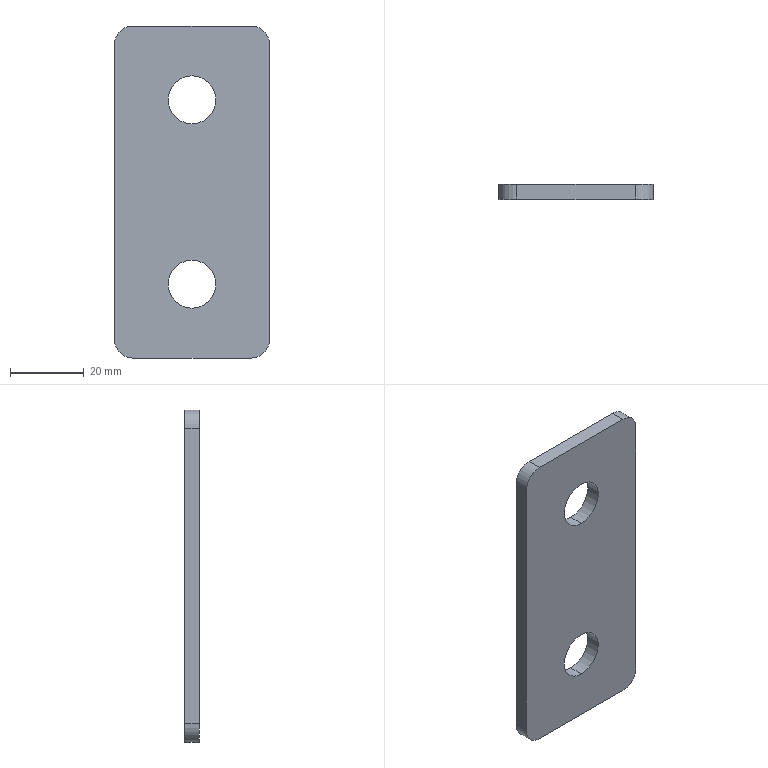Component | SolidWorks | ConnectingPlate(Item16)-1 | 1 solid | 14 faces | box 42 x 4 x 90 mm | volume 13972 mm3 | cylinder 8 | plane 6 | commonest cylinder face diameters 13 x4 10 x4 | material Plain Carbon Steel
STEP:
#1=COLOUR_RGB('',0.7922,0.8196,0.9333);
#2=FILL_AREA_STYLE_COLOUR('',#1);
#3=FILL_AREA_STYLE('',(#2));
#4=SURFACE_STYLE_FILL_AREA(#3);
#5=SURFACE_SIDE_STYLE('',(#4));
#6=SURFACE_STYLE_USAGE(.BOTH.,#5);
#7=PRESENTATION_STYLE_ASSIGNMENT((#6));
#8=CARTESIAN_POINT('',(14.764,14.843,-83.898));
#9=VERTEX_POINT('',#8);
#10=CARTESIAN_POINT('',(14.764,14.843,-84.409));
#11=VERTEX_POINT('',#10);
#12=CARTESIAN_POINT('',(14.764,14.843,-84.154));
#13=DIRECTION('',(-0.,1.,-0.));
#14=DIRECTION('',(0.,0.,1.));
#15=AXIS2_PLACEMENT_3D('',#12,#13,#14);
#16=CIRCLE('',#15,0.2559);
#17=EDGE_CURVE('',#9,#11,#16,.T.);
#18=ORIENTED_EDGE('',*,*,#17,.F.);
#19=CARTESIAN_POINT('',(14.764,15.,-83.898));
#20=VERTEX_POINT('',#19);
#21=CARTESIAN_POINT('',(14.764,14.843,-83.898));
#22=DIRECTION('',(-0.,1.,-0.));
#23=VECTOR('',#22,39.37);
#24=LINE('',#21,#23);
#25=EDGE_CURVE('',#9,#20,#24,.T.);
#26=ORIENTED_EDGE('',*,*,#25,.T.);
#27=CARTESIAN_POINT('',(14.764,15.,-84.409));
#28=VERTEX_POINT('',#27);
#29=CARTESIAN_POINT('',(14.764,15.,-84.154));
#30=DIRECTION('',(-0.,1.,-0.));
#31=DIRECTION('',(0.,0.,1.));
#32=AXIS2_PLACEMENT_3D('',#29,#30,#31);
#33=CIRCLE('',#32,0.2559);
#34=EDGE_CURVE('',#20,#28,#33,.T.);
#35=ORIENTED_EDGE('',*,*,#34,.T.);
#36=CARTESIAN_POINT('',(14.764,14.843,-84.409));
#37=DIRECTION('',(-0.,1.,-0.));
#38=VECTOR('',#37,39.37);
#39=LINE('',#36,#38);
#40=EDGE_CURVE('',#11,#28,#39,.T.);
#41=ORIENTED_EDGE('',*,*,#40,.F.);
#42=EDGE_LOOP('',(#18,#26,#35,#41));
#43=FACE_OUTER_BOUND('',#42,.T.);
#44=CARTESIAN_POINT('',(14.764,14.843,-84.154));
#45=DIRECTION('',(-0.,1.,-0.));
#46=DIRECTION('',(0.,0.,-1.));
#47=AXIS2_PLACEMENT_3D('',#44,#45,#46);
#48=CYLINDRICAL_SURFACE('',#47,0.2559);
#49=ADVANCED_FACE('',(#43),#48,.F.);
#50=CARTESIAN_POINT('',(14.764,14.843,-81.929));
#51=VERTEX_POINT('',#50);
#52=CARTESIAN_POINT('',(14.764,14.843,-82.441));
#53=VERTEX_POINT('',#52);
#54=CARTESIAN_POINT('',(14.764,14.843,-82.185));
#55=DIRECTION('',(-0.,1.,-0.));
#56=DIRECTION('',(0.,0.,-1.));
#57=AXIS2_PLACEMENT_3D('',#54,#55,#56);
#58=CIRCLE('',#57,0.2559);
#59=EDGE_CURVE('',#51,#53,#58,.T.);
#60=ORIENTED_EDGE('',*,*,#59,.F.);
#61=CARTESIAN_POINT('',(14.764,15.,-81.929));
#62=VERTEX_POINT('',#61);
#63=CARTESIAN_POINT('',(14.764,14.843,-81.929));
#64=DIRECTION('',(-0.,1.,-0.));
#65=VECTOR('',#64,39.37);
#66=LINE('',#63,#65);
#67=EDGE_CURVE('',#51,#62,#66,.T.);
#68=ORIENTED_EDGE('',*,*,#67,.T.);
#69=CARTESIAN_POINT('',(14.764,15.,-82.441));
#70=VERTEX_POINT('',#69);
#71=CARTESIAN_POINT('',(14.764,15.,-82.185));
#72=DIRECTION('',(-0.,1.,-0.));
#73=DIRECTION('',(0.,0.,-1.));
#74=AXIS2_PLACEMENT_3D('',#71,#72,#73);
#75=CIRCLE('',#74,0.2559);
#76=EDGE_CURVE('',#62,#70,#75,.T.);
#77=ORIENTED_EDGE('',*,*,#76,.T.);
#78=CARTESIAN_POINT('',(14.764,14.843,-82.441));
#79=DIRECTION('',(-0.,1.,-0.));
#80=VECTOR('',#79,39.37);
#81=LINE('',#78,#80);
#82=EDGE_CURVE('',#53,#70,#81,.T.);
#83=ORIENTED_EDGE('',*,*,#82,.F.);
#84=EDGE_LOOP('',(#60,#68,#77,#83));
#85=FACE_OUTER_BOUND('',#84,.T.);
#86=CARTESIAN_POINT('',(14.764,14.843,-82.185));
#87=DIRECTION('',(-0.,1.,-0.));
#88=DIRECTION('',(0.,0.,-1.));
#89=AXIS2_PLACEMENT_3D('',#86,#87,#88);
#90=CYLINDRICAL_SURFACE('',#89,0.2559);
#91=ADVANCED_FACE('',(#85),#90,.F.);
#92=CARTESIAN_POINT('',(15.394,15.,-84.941));
#93=VERTEX_POINT('',#92);
#94=CARTESIAN_POINT('',(14.134,15.,-84.941));
#95=VERTEX_POINT('',#94);
#96=CARTESIAN_POINT('',(15.591,15.,-84.941));
#97=DIRECTION('',(-1.,-0.,0.));
#98=VECTOR('',#97,39.37);
#99=LINE('',#96,#98);
#100=EDGE_CURVE('',#93,#95,#99,.T.);
#101=ORIENTED_EDGE('',*,*,#100,.F.);
#102=CARTESIAN_POINT('',(15.394,14.843,-84.941));
#103=VERTEX_POINT('',#102);
#104=CARTESIAN_POINT('',(15.394,14.843,-84.941));
#105=DIRECTION('',(0.,-1.,0.));
#106=VECTOR('',#105,39.37);
#107=LINE('',#104,#106);
#108=EDGE_CURVE('',#93,#103,#107,.T.);
#109=ORIENTED_EDGE('',*,*,#108,.T.);
#110=CARTESIAN_POINT('',(14.134,14.843,-84.941));
#111=VERTEX_POINT('',#110);
#112=CARTESIAN_POINT('',(15.591,14.843,-84.941));
#113=DIRECTION('',(-1.,-0.,0.));
#114=VECTOR('',#113,39.37);
#115=LINE('',#112,#114);
#116=EDGE_CURVE('',#103,#111,#115,.T.);
#117=ORIENTED_EDGE('',*,*,#116,.T.);
#118=CARTESIAN_POINT('',(14.134,14.843,-84.941));
#119=DIRECTION('',(-0.,1.,-0.));
#120=VECTOR('',#119,39.37);
#121=LINE('',#118,#120);
#122=EDGE_CURVE('',#111,#95,#121,.T.);
#123=ORIENTED_EDGE('',*,*,#122,.T.);
#124=EDGE_LOOP('',(#101,#109,#117,#123));
#125=FACE_OUTER_BOUND('',#124,.T.);
#126=CARTESIAN_POINT('',(15.591,14.843,-84.941));
#127=DIRECTION('',(-0.,-0.,-1.));
#128=DIRECTION('',(0.,-1.,0.));
#129=AXIS2_PLACEMENT_3D('',#126,#127,#128);
#130=PLANE('',#129);
#131=ADVANCED_FACE('',(#125),#130,.T.);
#132=CARTESIAN_POINT('',(15.591,15.,-81.594));
#133=VERTEX_POINT('',#132);
#134=CARTESIAN_POINT('',(15.591,15.,-84.744));
#135=VERTEX_POINT('',#134);
#136=CARTESIAN_POINT('',(15.591,15.,-81.398));
#137=DIRECTION('',(-0.,-0.,-1.));
#138=VECTOR('',#137,39.37);
#139=LINE('',#136,#138);
#140=EDGE_CURVE('',#133,#135,#139,.T.);
#141=ORIENTED_EDGE('',*,*,#140,.F.);
#142=CARTESIAN_POINT('',(15.591,14.843,-81.594));
#143=VERTEX_POINT('',#142);
#144=CARTESIAN_POINT('',(15.591,14.843,-81.594));
#145=DIRECTION('',(0.,-1.,0.));
#146=VECTOR('',#145,39.37);
#147=LINE('',#144,#146);
#148=EDGE_CURVE('',#133,#143,#147,.T.);
#149=ORIENTED_EDGE('',*,*,#148,.T.);
#150=CARTESIAN_POINT('',(15.591,14.843,-84.744));
#151=VERTEX_POINT('',#150);
#152=CARTESIAN_POINT('',(15.591,14.843,-81.398));
#153=DIRECTION('',(-0.,-0.,-1.));
#154=VECTOR('',#153,39.37);
#155=LINE('',#152,#154);
#156=EDGE_CURVE('',#143,#151,#155,.T.);
#157=ORIENTED_EDGE('',*,*,#156,.T.);
#158=CARTESIAN_POINT('',(15.591,14.843,-84.744));
#159=DIRECTION('',(-0.,1.,-0.));
#160=VECTOR('',#159,39.37);
#161=LINE('',#158,#160);
#162=EDGE_CURVE('',#151,#135,#161,.T.);
#163=ORIENTED_EDGE('',*,*,#162,.T.);
#164=EDGE_LOOP('',(#141,#149,#157,#163));
#165=FACE_OUTER_BOUND('',#164,.T.);
#166=CARTESIAN_POINT('',(15.591,14.843,-81.398));
#167=DIRECTION('',(1.,0.,-0.));
#168=DIRECTION('',(0.,-1.,0.));
#169=AXIS2_PLACEMENT_3D('',#166,#167,#168);
#170=PLANE('',#169);
#171=ADVANCED_FACE('',(#165),#170,.T.);
#172=CARTESIAN_POINT('',(14.134,14.843,-81.398));
#173=VERTEX_POINT('',#172);
#174=CARTESIAN_POINT('',(15.394,14.843,-81.398));
#175=VERTEX_POINT('',#174);
#176=CARTESIAN_POINT('',(15.591,14.843,-81.398));
#177=DIRECTION('',(1.,0.,-0.));
#178=VECTOR('',#177,39.37);
#179=LINE('',#176,#178);
#180=EDGE_CURVE('',#173,#175,#179,.T.);
#181=ORIENTED_EDGE('',*,*,#180,.T.);
#182=CARTESIAN_POINT('',(15.394,15.,-81.398));
#183=VERTEX_POINT('',#182);
#184=CARTESIAN_POINT('',(15.394,14.843,-81.398));
#185=DIRECTION('',(-0.,1.,-0.));
#186=VECTOR('',#185,39.37);
#187=LINE('',#184,#186);
#188=EDGE_CURVE('',#175,#183,#187,.T.);
#189=ORIENTED_EDGE('',*,*,#188,.T.);
#190=CARTESIAN_POINT('',(14.134,15.,-81.398));
#191=VERTEX_POINT('',#190);
#192=CARTESIAN_POINT('',(15.591,15.,-81.398));
#193=DIRECTION('',(1.,0.,-0.));
#194=VECTOR('',#193,39.37);
#195=LINE('',#192,#194);
#196=EDGE_CURVE('',#191,#183,#195,.T.);
#197=ORIENTED_EDGE('',*,*,#196,.F.);
#198=CARTESIAN_POINT('',(14.134,14.843,-81.398));
#199=DIRECTION('',(0.,-1.,0.));
#200=VECTOR('',#199,39.37);
#201=LINE('',#198,#200);
#202=EDGE_CURVE('',#191,#173,#201,.T.);
#203=ORIENTED_EDGE('',*,*,#202,.T.);
#204=EDGE_LOOP('',(#181,#189,#197,#203));
#205=FACE_OUTER_BOUND('',#204,.T.);
#206=CARTESIAN_POINT('',(15.591,14.843,-81.398));
#207=DIRECTION('',(0.,0.,1.));
#208=DIRECTION('',(-0.,1.,-0.));
#209=AXIS2_PLACEMENT_3D('',#206,#207,#208);
#210=PLANE('',#209);
#211=ADVANCED_FACE('',(#205),#210,.T.);
#212=CARTESIAN_POINT('',(13.937,14.843,-84.744));
#213=VERTEX_POINT('',#212);
#214=CARTESIAN_POINT('',(13.937,14.843,-81.594));
#215=VERTEX_POINT('',#214);
#216=CARTESIAN_POINT('',(13.937,14.843,-81.398));
#217=DIRECTION('',(0.,0.,1.));
#218=VECTOR('',#217,39.37);
#219=LINE('',#216,#218);
#220=EDGE_CURVE('',#213,#215,#219,.T.);
#221=ORIENTED_EDGE('',*,*,#220,.T.);
#222=CARTESIAN_POINT('',(13.937,15.,-81.594));
#223=VERTEX_POINT('',#222);
#224=CARTESIAN_POINT('',(13.937,14.843,-81.594));
#225=DIRECTION('',(-0.,1.,-0.));
#226=VECTOR('',#225,39.37);
#227=LINE('',#224,#226);
#228=EDGE_CURVE('',#215,#223,#227,.T.);
#229=ORIENTED_EDGE('',*,*,#228,.T.);
#230=CARTESIAN_POINT('',(13.937,15.,-84.744));
#231=VERTEX_POINT('',#230);
#232=CARTESIAN_POINT('',(13.937,15.,-81.398));
#233=DIRECTION('',(0.,0.,1.));
#234=VECTOR('',#233,39.37);
#235=LINE('',#232,#234);
#236=EDGE_CURVE('',#231,#223,#235,.T.);
#237=ORIENTED_EDGE('',*,*,#236,.F.);
#238=CARTESIAN_POINT('',(13.937,14.843,-84.744));
#239=DIRECTION('',(0.,-1.,0.));
#240=VECTOR('',#239,39.37);
#241=LINE('',#238,#240);
#242=EDGE_CURVE('',#231,#213,#241,.T.);
#243=ORIENTED_EDGE('',*,*,#242,.T.);
#244=EDGE_LOOP('',(#221,#229,#237,#243));
#245=FACE_OUTER_BOUND('',#244,.T.);
#246=CARTESIAN_POINT('',(13.937,14.843,-81.398));
#247=DIRECTION('',(-1.,-0.,0.));
#248=DIRECTION('',(-0.,1.,-0.));
#249=AXIS2_PLACEMENT_3D('',#246,#247,#248);
#250=PLANE('',#249);
#251=ADVANCED_FACE('',(#245),#250,.T.);
#252=CARTESIAN_POINT('',(14.764,14.843,-84.154));
#253=DIRECTION('',(-0.,1.,-0.));
#254=DIRECTION('',(0.,0.,1.));
#255=AXIS2_PLACEMENT_3D('',#252,#253,#254);
#256=CIRCLE('',#255,0.2559);
#257=EDGE_CURVE('',#11,#9,#256,.T.);
#258=ORIENTED_EDGE('',*,*,#257,.T.);
#259=ORIENTED_EDGE('',*,*,#17,.T.);
#260=EDGE_LOOP('',(#258,#259));
#261=FACE_BOUND('',#260,.T.);
#262=CARTESIAN_POINT('',(14.764,14.843,-82.185));
#263=DIRECTION('',(-0.,1.,-0.));
#264=DIRECTION('',(0.,0.,-1.));
#265=AXIS2_PLACEMENT_3D('',#262,#263,#264);
#266=CIRCLE('',#265,0.2559);
#267=EDGE_CURVE('',#53,#51,#266,.T.);
#268=ORIENTED_EDGE('',*,*,#267,.T.);
#269=ORIENTED_EDGE('',*,*,#59,.T.);
#270=EDGE_LOOP('',(#268,#269));
#271=FACE_BOUND('',#270,.T.);
#272=ORIENTED_EDGE('',*,*,#156,.F.);
#273=CARTESIAN_POINT('',(15.394,14.843,-81.594));
#274=DIRECTION('',(0.,-1.,0.));
#275=DIRECTION('',(0.,0.,1.));
#276=AXIS2_PLACEMENT_3D('',#273,#274,#275);
#277=CIRCLE('',#276,0.1969);
#278=EDGE_CURVE('',#143,#175,#277,.T.);
#279=ORIENTED_EDGE('',*,*,#278,.T.);
#280=ORIENTED_EDGE('',*,*,#180,.F.);
#281=CARTESIAN_POINT('',(14.134,14.843,-81.594));
#282=DIRECTION('',(0.,-1.,0.));
#283=DIRECTION('',(0.,0.,1.));
#284=AXIS2_PLACEMENT_3D('',#281,#282,#283);
#285=CIRCLE('',#284,0.1969);
#286=EDGE_CURVE('',#173,#215,#285,.T.);
#287=ORIENTED_EDGE('',*,*,#286,.T.);
#288=ORIENTED_EDGE('',*,*,#220,.F.);
#289=CARTESIAN_POINT('',(14.134,14.843,-84.744));
#290=DIRECTION('',(0.,-1.,0.));
#291=DIRECTION('',(0.,0.,1.));
#292=AXIS2_PLACEMENT_3D('',#289,#290,#291);
#293=CIRCLE('',#292,0.1969);
#294=EDGE_CURVE('',#213,#111,#293,.T.);
#295=ORIENTED_EDGE('',*,*,#294,.T.);
#296=ORIENTED_EDGE('',*,*,#116,.F.);
#297=CARTESIAN_POINT('',(15.394,14.843,-84.744));
#298=DIRECTION('',(0.,-1.,0.));
#299=DIRECTION('',(0.,0.,1.));
#300=AXIS2_PLACEMENT_3D('',#297,#298,#299);
#301=CIRCLE('',#300,0.1969);
#302=EDGE_CURVE('',#103,#151,#301,.T.);
#303=ORIENTED_EDGE('',*,*,#302,.T.);
#304=EDGE_LOOP('',(#272,#279,#280,#287,#288,#295,#296,#303));
#305=FACE_OUTER_BOUND('',#304,.T.);
#306=CARTESIAN_POINT('',(13.937,14.843,-84.941));
#307=DIRECTION('',(0.,-1.,0.));
#308=DIRECTION('',(0.,0.,1.));
#309=AXIS2_PLACEMENT_3D('',#306,#307,#308);
#310=PLANE('',#309);
#311=ADVANCED_FACE('',(#261,#271,#305),#310,.T.);
#312=CARTESIAN_POINT('',(14.764,15.,-84.154));
#313=DIRECTION('',(-0.,1.,-0.));
#314=DIRECTION('',(0.,0.,1.));
#315=AXIS2_PLACEMENT_3D('',#312,#313,#314);
#316=CIRCLE('',#315,0.2559);
#317=EDGE_CURVE('',#28,#20,#316,.T.);
#318=ORIENTED_EDGE('',*,*,#317,.F.);
#319=ORIENTED_EDGE('',*,*,#34,.F.);
#320=EDGE_LOOP('',(#318,#319));
#321=FACE_BOUND('',#320,.T.);
#322=CARTESIAN_POINT('',(14.764,15.,-82.185));
#323=DIRECTION('',(-0.,1.,-0.));
#324=DIRECTION('',(0.,0.,-1.));
#325=AXIS2_PLACEMENT_3D('',#322,#323,#324);
#326=CIRCLE('',#325,0.2559);
#327=EDGE_CURVE('',#70,#62,#326,.T.);
#328=ORIENTED_EDGE('',*,*,#327,.F.);
#329=ORIENTED_EDGE('',*,*,#76,.F.);
#330=EDGE_LOOP('',(#328,#329));
#331=FACE_BOUND('',#330,.T.);
#332=ORIENTED_EDGE('',*,*,#196,.T.);
#333=CARTESIAN_POINT('',(15.394,15.,-81.594));
#334=DIRECTION('',(-0.,1.,-0.));
#335=DIRECTION('',(0.,0.,1.));
#336=AXIS2_PLACEMENT_3D('',#333,#334,#335);
#337=CIRCLE('',#336,0.1969);
#338=EDGE_CURVE('',#183,#133,#337,.T.);
#339=ORIENTED_EDGE('',*,*,#338,.T.);
#340=ORIENTED_EDGE('',*,*,#140,.T.);
#341=CARTESIAN_POINT('',(15.394,15.,-84.744));
#342=DIRECTION('',(-0.,1.,-0.));
#343=DIRECTION('',(0.,0.,1.));
#344=AXIS2_PLACEMENT_3D('',#341,#342,#343);
#345=CIRCLE('',#344,0.1969);
#346=EDGE_CURVE('',#135,#93,#345,.T.);
#347=ORIENTED_EDGE('',*,*,#346,.T.);
#348=ORIENTED_EDGE('',*,*,#100,.T.);
#349=CARTESIAN_POINT('',(14.134,15.,-84.744));
#350=DIRECTION('',(-0.,1.,-0.));
#351=DIRECTION('',(0.,0.,1.));
#352=AXIS2_PLACEMENT_3D('',#349,#350,#351);
#353=CIRCLE('',#352,0.1969);
#354=EDGE_CURVE('',#95,#231,#353,.T.);
#355=ORIENTED_EDGE('',*,*,#354,.T.);
#356=ORIENTED_EDGE('',*,*,#236,.T.);
#357=CARTESIAN_POINT('',(14.134,15.,-81.594));
#358=DIRECTION('',(-0.,1.,-0.));
#359=DIRECTION('',(0.,0.,1.));
#360=AXIS2_PLACEMENT_3D('',#357,#358,#359);
#361=CIRCLE('',#360,0.1969);
#362=EDGE_CURVE('',#223,#191,#361,.T.);
#363=ORIENTED_EDGE('',*,*,#362,.T.);
#364=EDGE_LOOP('',(#332,#339,#340,#347,#348,#355,#356,#363));
#365=FACE_OUTER_BOUND('',#364,.T.);
#366=CARTESIAN_POINT('',(13.937,15.,-84.941));
#367=DIRECTION('',(0.,-1.,0.));
#368=DIRECTION('',(0.,0.,1.));
#369=AXIS2_PLACEMENT_3D('',#366,#367,#368);
#370=PLANE('',#369);
#371=ADVANCED_FACE('',(#321,#331,#365),#370,.F.);
#372=ORIENTED_EDGE('',*,*,#67,.F.);
#373=ORIENTED_EDGE('',*,*,#267,.F.);
#374=ORIENTED_EDGE('',*,*,#82,.T.);
#375=ORIENTED_EDGE('',*,*,#327,.T.);
#376=EDGE_LOOP('',(#372,#373,#374,#375));
#377=FACE_OUTER_BOUND('',#376,.T.);
#378=CARTESIAN_POINT('',(14.764,14.843,-82.185));
#379=DIRECTION('',(-0.,1.,-0.));
#380=DIRECTION('',(0.,0.,-1.));
#381=AXIS2_PLACEMENT_3D('',#378,#379,#380);
#382=CYLINDRICAL_SURFACE('',#381,0.2559);
#383=ADVANCED_FACE('',(#377),#382,.F.);
#384=ORIENTED_EDGE('',*,*,#25,.F.);
#385=ORIENTED_EDGE('',*,*,#257,.F.);
#386=ORIENTED_EDGE('',*,*,#40,.T.);
#387=ORIENTED_EDGE('',*,*,#317,.T.);
#388=EDGE_LOOP('',(#384,#385,#386,#387));
#389=FACE_OUTER_BOUND('',#388,.T.);
#390=CARTESIAN_POINT('',(14.764,14.843,-84.154));
#391=DIRECTION('',(-0.,1.,-0.));
#392=DIRECTION('',(0.,0.,-1.));
#393=AXIS2_PLACEMENT_3D('',#390,#391,#392);
#394=CYLINDRICAL_SURFACE('',#393,0.2559);
#395=ADVANCED_FACE('',(#389),#394,.F.);
#396=ORIENTED_EDGE('',*,*,#278,.F.);
#397=ORIENTED_EDGE('',*,*,#148,.F.);
#398=ORIENTED_EDGE('',*,*,#338,.F.);
#399=ORIENTED_EDGE('',*,*,#188,.F.);
#400=EDGE_LOOP('',(#396,#397,#398,#399));
#401=FACE_OUTER_BOUND('',#400,.T.);
#402=CARTESIAN_POINT('',(15.394,14.843,-81.594));
#403=DIRECTION('',(-0.,1.,-0.));
#404=DIRECTION('',(0.,0.,-1.));
#405=AXIS2_PLACEMENT_3D('',#402,#403,#404);
#406=CYLINDRICAL_SURFACE('',#405,0.1969);
#407=ADVANCED_FACE('',(#401),#406,.T.);
#408=ORIENTED_EDGE('',*,*,#286,.F.);
#409=ORIENTED_EDGE('',*,*,#202,.F.);
#410=ORIENTED_EDGE('',*,*,#362,.F.);
#411=ORIENTED_EDGE('',*,*,#228,.F.);
#412=EDGE_LOOP('',(#408,#409,#410,#411));
#413=FACE_OUTER_BOUND('',#412,.T.);
#414=CARTESIAN_POINT('',(14.134,14.843,-81.594));
#415=DIRECTION('',(-0.,1.,-0.));
#416=DIRECTION('',(0.,0.,-1.));
#417=AXIS2_PLACEMENT_3D('',#414,#415,#416);
#418=CYLINDRICAL_SURFACE('',#417,0.1969);
#419=ADVANCED_FACE('',(#413),#418,.T.);
#420=ORIENTED_EDGE('',*,*,#302,.F.);
#421=ORIENTED_EDGE('',*,*,#108,.F.);
#422=ORIENTED_EDGE('',*,*,#346,.F.);
#423=ORIENTED_EDGE('',*,*,#162,.F.);
#424=EDGE_LOOP('',(#420,#421,#422,#423));
#425=FACE_OUTER_BOUND('',#424,.T.);
#426=CARTESIAN_POINT('',(15.394,14.843,-84.744));
#427=DIRECTION('',(-0.,1.,-0.));
#428=DIRECTION('',(0.,0.,-1.));
#429=AXIS2_PLACEMENT_3D('',#426,#427,#428);
#430=CYLINDRICAL_SURFACE('',#429,0.1969);
#431=ADVANCED_FACE('',(#425),#430,.T.);
#432=ORIENTED_EDGE('',*,*,#294,.F.);
#433=ORIENTED_EDGE('',*,*,#242,.F.);
#434=ORIENTED_EDGE('',*,*,#354,.F.);
#435=ORIENTED_EDGE('',*,*,#122,.F.);
#436=EDGE_LOOP('',(#432,#433,#434,#435));
#437=FACE_OUTER_BOUND('',#436,.T.);
#438=CARTESIAN_POINT('',(14.134,14.843,-84.744));
#439=DIRECTION('',(-0.,1.,-0.));
#440=DIRECTION('',(0.,0.,-1.));
#441=AXIS2_PLACEMENT_3D('',#438,#439,#440);
#442=CYLINDRICAL_SURFACE('',#441,0.1969);
#443=ADVANCED_FACE('',(#437),#442,.T.);
#444=CLOSED_SHELL('',(#49,#91,#131,#171,#211,#251,#311,#371,#383,#395,#407,#419,#431,#443));
#445=MANIFOLD_SOLID_BREP('',#444);
#446=STYLED_ITEM('',(#7),#445);
#447=PRESENTATION_LAYER_ASSIGNMENT('','',(#446));
#448=CARTESIAN_POINT('',(0.,0.,0.));
#449=DIRECTION('',(0.,0.,1.));
#450=DIRECTION('',(1.,0.,0.));
#451=AXIS2_PLACEMENT_3D('',#448,#449,#450);
#452=(LENGTH_UNIT()NAMED_UNIT(*)SI_UNIT($,.METRE.));
#453=LENGTH_MEASURE_WITH_UNIT(LENGTH_MEASURE(0.0254),#452);
#454=DIMENSIONAL_EXPONENTS(1.,0.,0.,0.,0.,0.,0.);
#455=(CONVERSION_BASED_UNIT('',#453)LENGTH_UNIT()NAMED_UNIT(#454));
#456=UNCERTAINTY_MEASURE_WITH_UNIT(LENGTH_MEASURE(0.00001),#455,'','');
#457=(NAMED_UNIT(*)PLANE_ANGLE_UNIT()SI_UNIT($,.RADIAN.));
#458=(NAMED_UNIT(*)SI_UNIT($,.STERADIAN.)SOLID_ANGLE_UNIT());
#459=(GEOMETRIC_REPRESENTATION_CONTEXT(3)GLOBAL_UNCERTAINTY_ASSIGNED_CONTEXT((#456))GLOBAL_UNIT_ASSIGNED_CONTEXT((#455,#457,#458))REPRESENTATION_CONTEXT('',''));
#460=ADVANCED_BREP_SHAPE_REPRESENTATION('',(#445,#451),#459);
#461=(LENGTH_UNIT()NAMED_UNIT(*)SI_UNIT($,.METRE.));
#462=LENGTH_MEASURE_WITH_UNIT(LENGTH_MEASURE(0.0254),#461);
#463=DIMENSIONAL_EXPONENTS(1.,0.,0.,0.,0.,0.,0.);
#464=(CONVERSION_BASED_UNIT('',#462)LENGTH_UNIT()NAMED_UNIT(#463));
#465=UNCERTAINTY_MEASURE_WITH_UNIT(LENGTH_MEASURE(0.00001),#464,'','');
#466=(NAMED_UNIT(*)PLANE_ANGLE_UNIT()SI_UNIT($,.RADIAN.));
#467=(NAMED_UNIT(*)SI_UNIT($,.STERADIAN.)SOLID_ANGLE_UNIT());
#468=(GEOMETRIC_REPRESENTATION_CONTEXT(3)GLOBAL_UNCERTAINTY_ASSIGNED_CONTEXT((#465))GLOBAL_UNIT_ASSIGNED_CONTEXT((#464,#466,#467))REPRESENTATION_CONTEXT('',''));
#469=MECHANICAL_DESIGN_GEOMETRIC_PRESENTATION_REPRESENTATION('',(#446),#468);